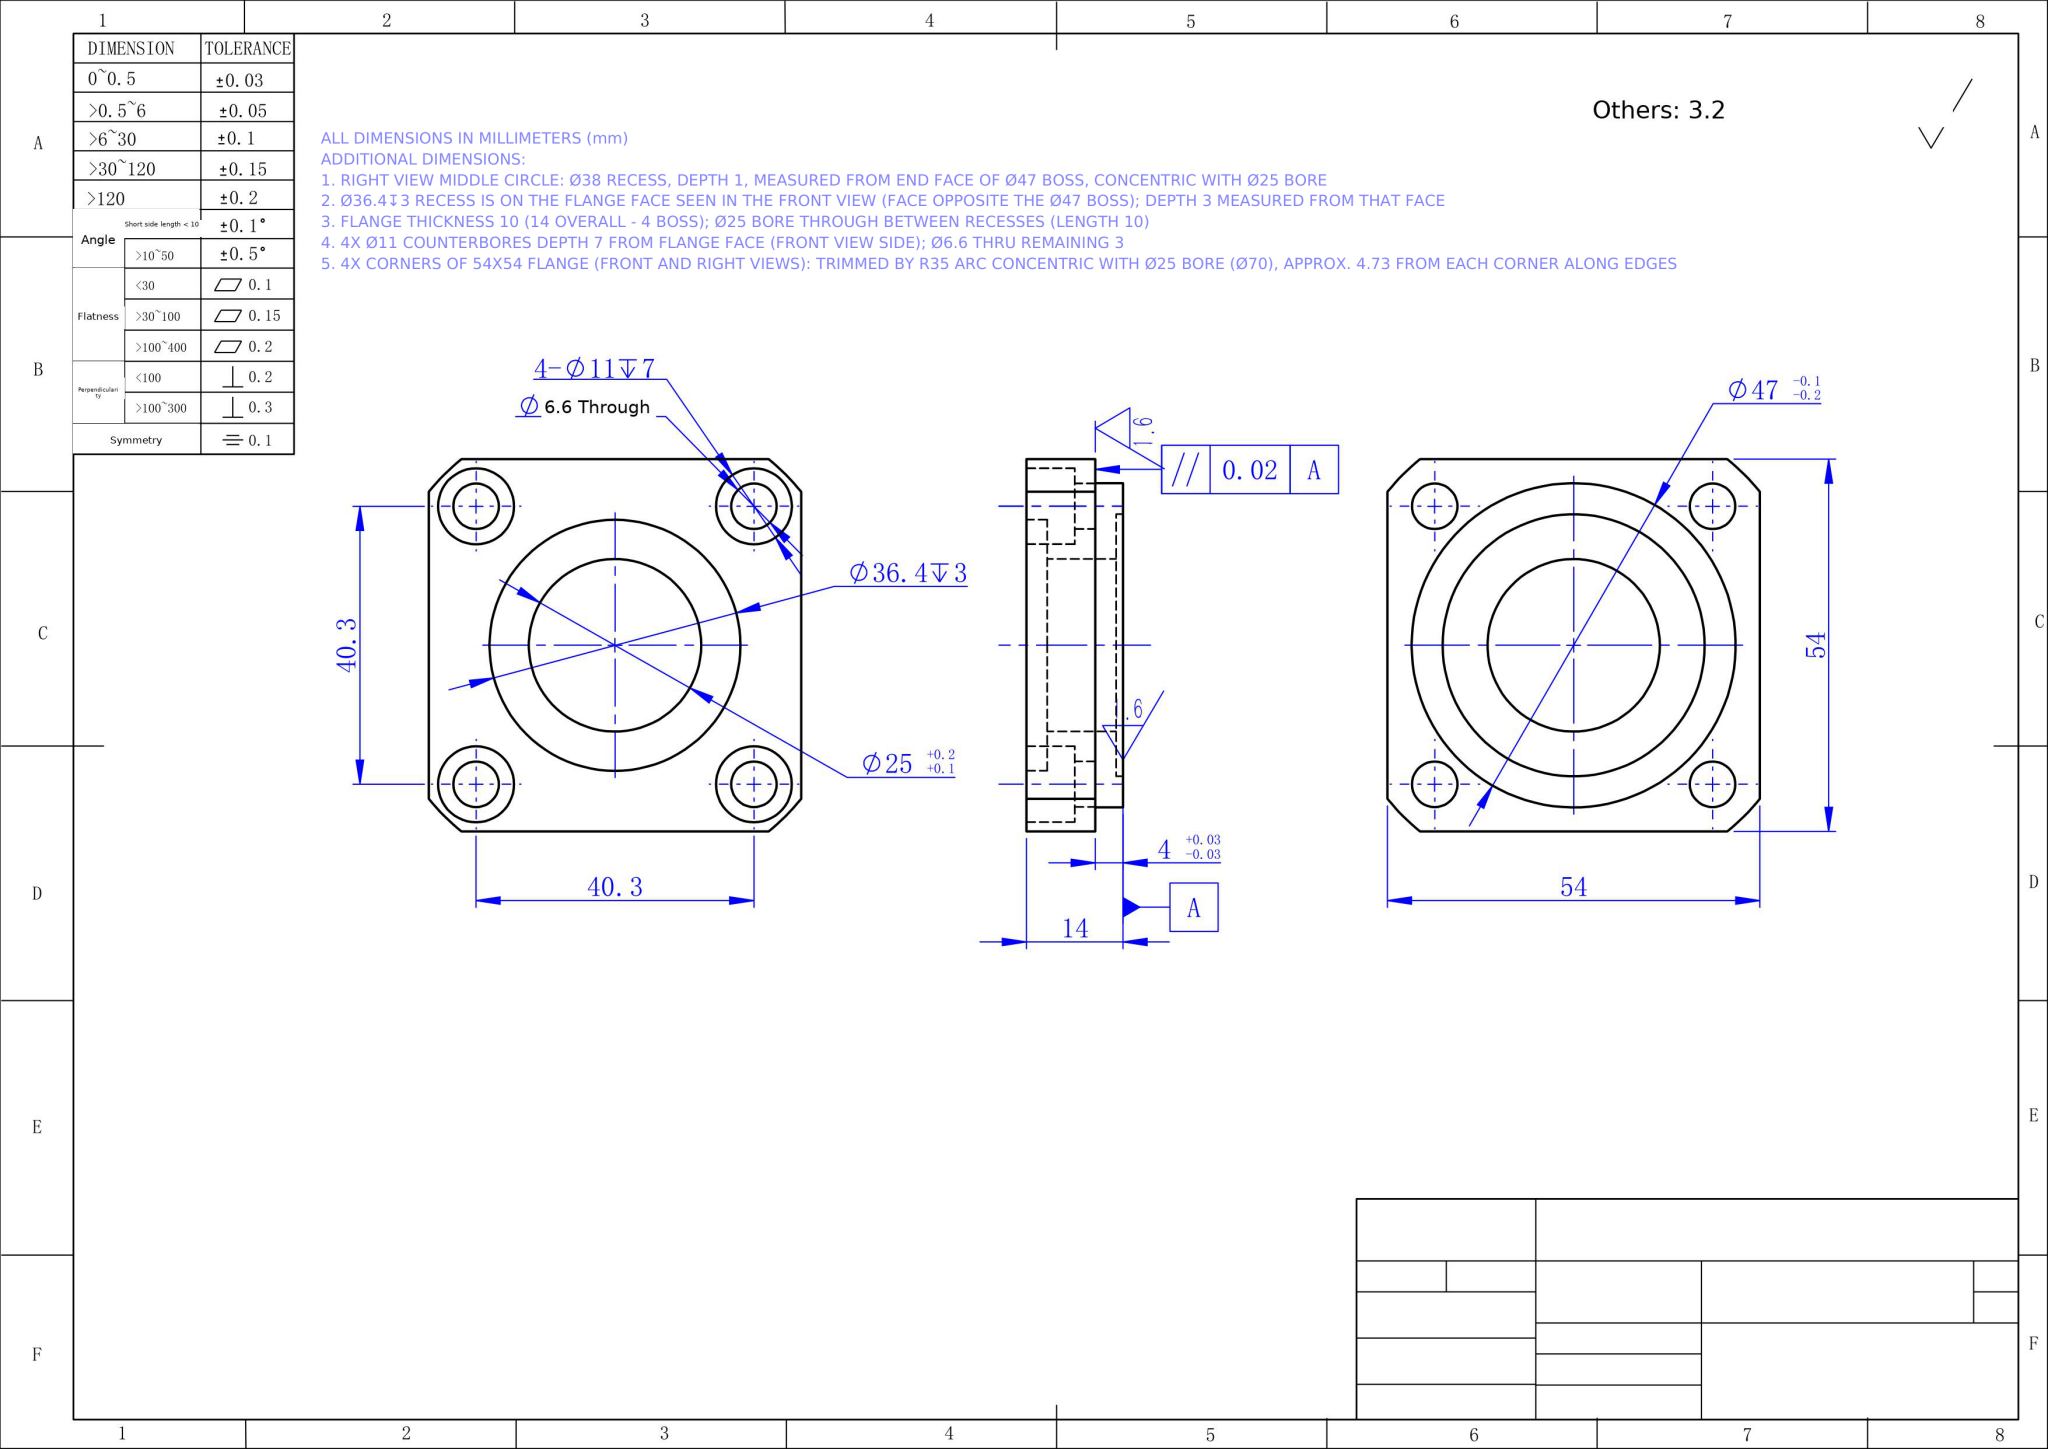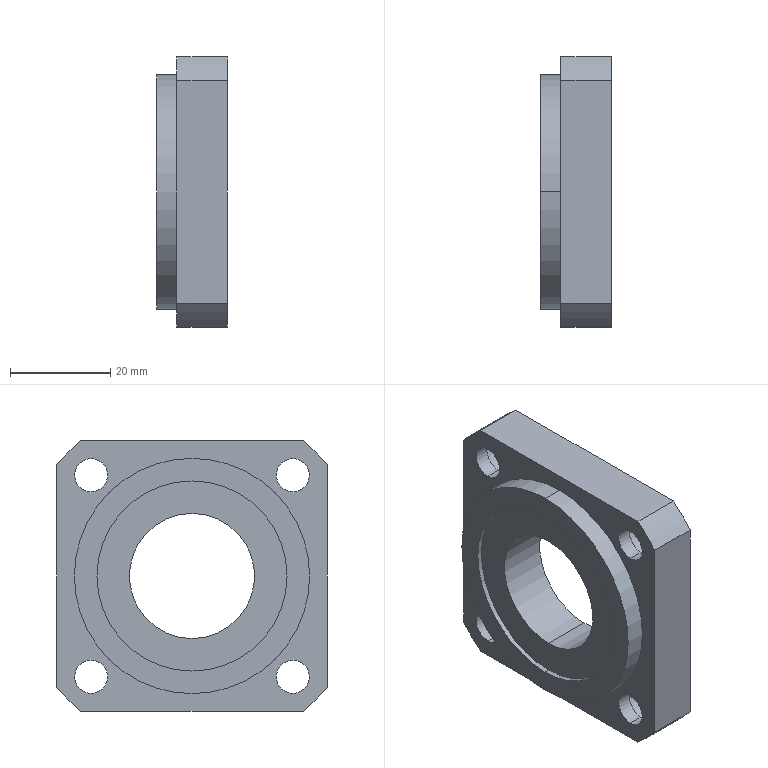Part | NX | mm | 1 solid | 41 faces | box 14 x 54 x 54 mm | volume 23445 mm3 | cylinder 28 | plane 13 | commonest cylinder face diameters 6.6 x8 11 x8 70 x4 38 x2 36.4 x2 47 x2 25 x2